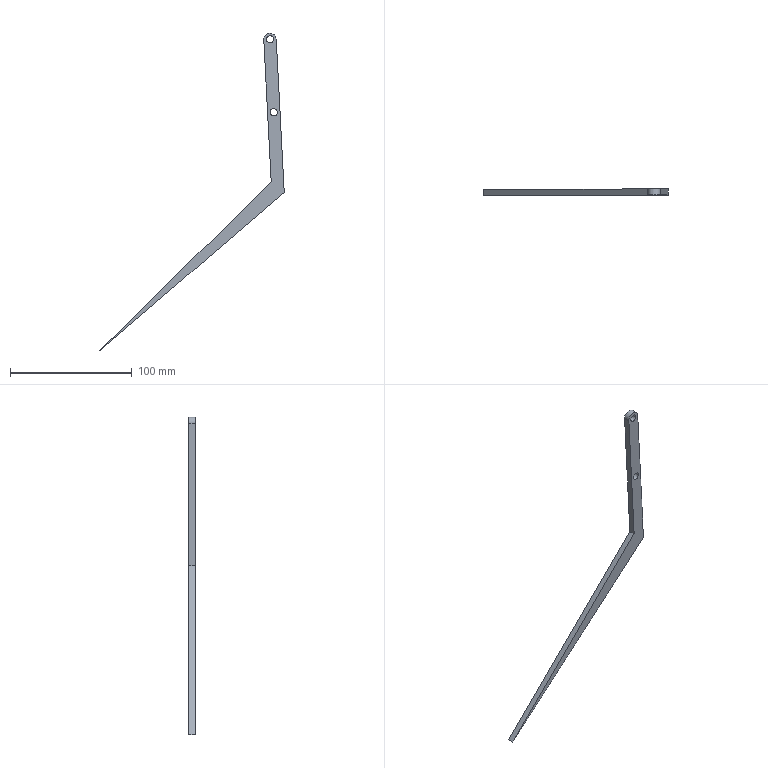Component | NX | 60 | 1 solid | 9 faces | box 151.75 x 5 x 261.36 mm | volume 12968 mm3 | plane 6 | cylinder 3 | commonest cylinder face diameters 5.929 x2 10.285 x1
STEP:
#1=CARTESIAN_POINT('',(0.,0.,0.));
#2=DIRECTION('',(0.,0.,1.));
#3=DIRECTION('',(1.,0.,0.));
#4=AXIS2_PLACEMENT_3D('',#1,#2,#3);
#5=CARTESIAN_POINT('',(-509.855,45.95,59.65));
#6=VERTEX_POINT('',#5);
#7=CARTESIAN_POINT('',(-499.584,45.95,60.187));
#8=VERTEX_POINT('',#7);
#9=CARTESIAN_POINT('',(-504.719,45.95,59.918));
#10=DIRECTION('',(0.,1.,0.));
#11=DIRECTION('',(-0.9986,0.,-0.05219));
#12=AXIS2_PLACEMENT_3D('',#9,#10,#11);
#13=CIRCLE('',#12,5.142);
#14=CARTESIAN_POINT('',(-504.719,40.95,59.918));
#15=DIRECTION('',(0.,1.,0.));
#16=DIRECTION('',(-0.9986,0.,-0.05219));
#17=AXIS2_PLACEMENT_3D('',#14,#15,#16);
#18=CYLINDRICAL_SURFACE('',#17,5.142);
#19=CARTESIAN_POINT('',(0.,5.));
#20=DIRECTION('',(1.,0.));
#21=VECTOR('',#20,1.);
#22=LINE('',#19,#21);
#23=(GEOMETRIC_REPRESENTATION_CONTEXT(2)PARAMETRIC_REPRESENTATION_CONTEXT()REPRESENTATION_CONTEXT('',''));
#24=DEFINITIONAL_REPRESENTATION('',(#22),#23);
#25=PCURVE('',#18,#24);
#26=CARTESIAN_POINT('',(-504.719,45.95,59.918));
#27=DIRECTION('',(0.,1.,0.));
#28=DIRECTION('',(-0.9986,0.,-0.05219));
#29=AXIS2_PLACEMENT_3D('',#26,#27,#28);
#30=PLANE('',#29);
#31=CARTESIAN_POINT('',(0.,0.));
#32=DIRECTION('',(1.,-0.));
#33=AXIS2_PLACEMENT_2D('',#31,#32);
#34=CIRCLE('',#33,5.142);
#35=(GEOMETRIC_REPRESENTATION_CONTEXT(2)PARAMETRIC_REPRESENTATION_CONTEXT()REPRESENTATION_CONTEXT('',''));
#36=DEFINITIONAL_REPRESENTATION('',(#34),#35);
#37=PCURVE('',#30,#36);
#38=SURFACE_CURVE('',#13,(#25,#37),.PCURVE_S1.);
#39=EDGE_CURVE('',#6,#8,#38,.T.);
#40=ORIENTED_EDGE('',*,*,#39,.F.);
#41=CARTESIAN_POINT('',(-509.855,40.95,59.65));
#42=VERTEX_POINT('',#41);
#43=CARTESIAN_POINT('',(-509.855,40.95,59.65));
#44=DIRECTION('',(0.,1.,0.));
#45=VECTOR('',#44,1.);
#46=LINE('',#43,#45);
#47=CARTESIAN_POINT('',(0.,0.));
#48=DIRECTION('',(0.,1.));
#49=VECTOR('',#48,1.);
#50=LINE('',#47,#49);
#51=(GEOMETRIC_REPRESENTATION_CONTEXT(2)PARAMETRIC_REPRESENTATION_CONTEXT()REPRESENTATION_CONTEXT('',''));
#52=DEFINITIONAL_REPRESENTATION('',(#50),#51);
#53=PCURVE('',#18,#52);
#54=CARTESIAN_POINT('',(-503.751,40.95,-57.127));
#55=DIRECTION('',(-0.9986,0.,-0.05219));
#56=DIRECTION('',(-0.05219,0.,0.9986));
#57=AXIS2_PLACEMENT_3D('',#54,#55,#56);
#58=PLANE('',#57);
#59=CARTESIAN_POINT('',(116.936,0.));
#60=DIRECTION('',(0.,1.));
#61=VECTOR('',#60,1.);
#62=LINE('',#59,#61);
#63=(GEOMETRIC_REPRESENTATION_CONTEXT(2)PARAMETRIC_REPRESENTATION_CONTEXT()REPRESENTATION_CONTEXT('',''));
#64=DEFINITIONAL_REPRESENTATION('',(#62),#63);
#65=PCURVE('',#58,#64);
#66=SURFACE_CURVE('',#46,(#53,#65),.PCURVE_S1.);
#67=EDGE_CURVE('',#42,#6,#66,.T.);
#68=ORIENTED_EDGE('',*,*,#67,.F.);
#69=CARTESIAN_POINT('',(-499.584,40.95,60.187));
#70=VERTEX_POINT('',#69);
#71=CARTESIAN_POINT('',(-504.719,40.95,59.918));
#72=DIRECTION('',(0.,1.,0.));
#73=DIRECTION('',(-0.9986,0.,-0.05219));
#74=AXIS2_PLACEMENT_3D('',#71,#72,#73);
#75=CIRCLE('',#74,5.142);
#76=CARTESIAN_POINT('',(0.,0.));
#77=DIRECTION('',(1.,0.));
#78=VECTOR('',#77,1.);
#79=LINE('',#76,#78);
#80=(GEOMETRIC_REPRESENTATION_CONTEXT(2)PARAMETRIC_REPRESENTATION_CONTEXT()REPRESENTATION_CONTEXT('',''));
#81=DEFINITIONAL_REPRESENTATION('',(#79),#80);
#82=PCURVE('',#18,#81);
#83=CARTESIAN_POINT('',(-504.719,40.95,59.918));
#84=DIRECTION('',(0.,1.,0.));
#85=DIRECTION('',(-0.9986,0.,-0.05219));
#86=AXIS2_PLACEMENT_3D('',#83,#84,#85);
#87=PLANE('',#86);
#88=CARTESIAN_POINT('',(0.,0.));
#89=DIRECTION('',(1.,-0.));
#90=AXIS2_PLACEMENT_2D('',#88,#89);
#91=CIRCLE('',#90,5.142);
#92=(GEOMETRIC_REPRESENTATION_CONTEXT(2)PARAMETRIC_REPRESENTATION_CONTEXT()REPRESENTATION_CONTEXT('',''));
#93=DEFINITIONAL_REPRESENTATION('',(#91),#92);
#94=PCURVE('',#87,#93);
#95=SURFACE_CURVE('',#75,(#82,#94),.PCURVE_S1.);
#96=EDGE_CURVE('',#42,#70,#95,.T.);
#97=ORIENTED_EDGE('',*,*,#96,.T.);
#98=CARTESIAN_POINT('',(-499.584,40.95,60.187));
#99=DIRECTION('',(0.,1.,0.));
#100=VECTOR('',#99,1.);
#101=LINE('',#98,#100);
#102=CARTESIAN_POINT('',(3.142,0.));
#103=DIRECTION('',(0.,1.));
#104=VECTOR('',#103,1.);
#105=LINE('',#102,#104);
#106=(GEOMETRIC_REPRESENTATION_CONTEXT(2)PARAMETRIC_REPRESENTATION_CONTEXT()REPRESENTATION_CONTEXT('',''));
#107=DEFINITIONAL_REPRESENTATION('',(#105),#106);
#108=PCURVE('',#18,#107);
#109=CARTESIAN_POINT('',(-496.452,40.95,0.2684));
#110=DIRECTION('',(0.9986,0.,0.05219));
#111=DIRECTION('',(0.05219,0.,-0.9986));
#112=AXIS2_PLACEMENT_3D('',#109,#110,#111);
#113=PLANE('',#112);
#114=CARTESIAN_POINT('',(-60.,0.));
#115=DIRECTION('',(0.,1.));
#116=VECTOR('',#115,1.);
#117=LINE('',#114,#116);
#118=(GEOMETRIC_REPRESENTATION_CONTEXT(2)PARAMETRIC_REPRESENTATION_CONTEXT()REPRESENTATION_CONTEXT('',''));
#119=DEFINITIONAL_REPRESENTATION('',(#117),#118);
#120=PCURVE('',#113,#119);
#121=SURFACE_CURVE('',#101,(#108,#120),.PCURVE_S1.);
#122=EDGE_CURVE('',#70,#8,#121,.T.);
#123=ORIENTED_EDGE('',*,*,#122,.T.);
#124=EDGE_LOOP('',(#40,#68,#97,#123));
#125=FACE_BOUND('',#124,.T.);
#126=ADVANCED_FACE('',(#125),#18,.T.);
#127=CARTESIAN_POINT('',(-493.001,45.95,-65.77));
#128=VERTEX_POINT('',#127);
#129=CARTESIAN_POINT('',(-496.452,45.95,0.2684));
#130=DIRECTION('',(0.05219,0.,-0.9986));
#131=VECTOR('',#130,1.);
#132=LINE('',#129,#131);
#133=CARTESIAN_POINT('',(0.,5.));
#134=DIRECTION('',(1.,0.));
#135=VECTOR('',#134,1.);
#136=LINE('',#133,#135);
#137=(GEOMETRIC_REPRESENTATION_CONTEXT(2)PARAMETRIC_REPRESENTATION_CONTEXT()REPRESENTATION_CONTEXT('',''));
#138=DEFINITIONAL_REPRESENTATION('',(#136),#137);
#139=PCURVE('',#113,#138);
#140=CARTESIAN_POINT('',(-5.142,-60.));
#141=DIRECTION('',(0.,-1.));
#142=VECTOR('',#141,1.);
#143=LINE('',#140,#142);
#144=(GEOMETRIC_REPRESENTATION_CONTEXT(2)PARAMETRIC_REPRESENTATION_CONTEXT()REPRESENTATION_CONTEXT('',''));
#145=DEFINITIONAL_REPRESENTATION('',(#143),#144);
#146=PCURVE('',#30,#145);
#147=SURFACE_CURVE('',#132,(#139,#146),.PCURVE_S1.);
#148=EDGE_CURVE('',#8,#128,#147,.T.);
#149=ORIENTED_EDGE('',*,*,#148,.F.);
#150=ORIENTED_EDGE('',*,*,#122,.F.);
#151=CARTESIAN_POINT('',(-493.001,40.95,-65.77));
#152=VERTEX_POINT('',#151);
#153=CARTESIAN_POINT('',(-499.584,40.95,60.187));
#154=DIRECTION('',(0.05219,0.,-0.9986));
#155=VECTOR('',#154,1.);
#156=LINE('',#153,#155);
#157=CARTESIAN_POINT('',(-60.,0.));
#158=DIRECTION('',(1.,0.));
#159=VECTOR('',#158,1.);
#160=LINE('',#157,#159);
#161=(GEOMETRIC_REPRESENTATION_CONTEXT(2)PARAMETRIC_REPRESENTATION_CONTEXT()REPRESENTATION_CONTEXT('',''));
#162=DEFINITIONAL_REPRESENTATION('',(#160),#161);
#163=PCURVE('',#113,#162);
#164=CARTESIAN_POINT('',(-5.142,0.));
#165=DIRECTION('',(0.,-1.));
#166=VECTOR('',#165,1.);
#167=LINE('',#164,#166);
#168=(GEOMETRIC_REPRESENTATION_CONTEXT(2)PARAMETRIC_REPRESENTATION_CONTEXT()REPRESENTATION_CONTEXT('',''));
#169=DEFINITIONAL_REPRESENTATION('',(#167),#168);
#170=PCURVE('',#87,#169);
#171=SURFACE_CURVE('',#156,(#163,#170),.PCURVE_S1.);
#172=EDGE_CURVE('',#70,#152,#171,.T.);
#173=ORIENTED_EDGE('',*,*,#172,.T.);
#174=CARTESIAN_POINT('',(-493.001,40.95,-65.77));
#175=DIRECTION('',(0.,1.,0.));
#176=VECTOR('',#175,1.);
#177=LINE('',#174,#176);
#178=CARTESIAN_POINT('',(66.128,0.));
#179=DIRECTION('',(0.,1.));
#180=VECTOR('',#179,1.);
#181=LINE('',#178,#180);
#182=(GEOMETRIC_REPRESENTATION_CONTEXT(2)PARAMETRIC_REPRESENTATION_CONTEXT()REPRESENTATION_CONTEXT('',''));
#183=DEFINITIONAL_REPRESENTATION('',(#181),#182);
#184=PCURVE('',#113,#183);
#185=CARTESIAN_POINT('',(-493.001,40.95,-65.77));
#186=DIRECTION('',(0.6521,0.,-0.7581));
#187=DIRECTION('',(-0.7581,0.,-0.6521));
#188=AXIS2_PLACEMENT_3D('',#185,#186,#187);
#189=PLANE('',#188);
#190=CARTESIAN_POINT('',(0.,0.));
#191=DIRECTION('',(0.,1.));
#192=VECTOR('',#191,1.);
#193=LINE('',#190,#192);
#194=(GEOMETRIC_REPRESENTATION_CONTEXT(2)PARAMETRIC_REPRESENTATION_CONTEXT()REPRESENTATION_CONTEXT('',''));
#195=DEFINITIONAL_REPRESENTATION('',(#193),#194);
#196=PCURVE('',#189,#195);
#197=SURFACE_CURVE('',#177,(#184,#196),.PCURVE_S1.);
#198=EDGE_CURVE('',#152,#128,#197,.T.);
#199=ORIENTED_EDGE('',*,*,#198,.T.);
#200=EDGE_LOOP('',(#149,#150,#173,#199));
#201=FACE_BOUND('',#200,.T.);
#202=ADVANCED_FACE('',(#201),#113,.T.);
#203=CARTESIAN_POINT('',(-644.746,45.95,-196.297));
#204=VERTEX_POINT('',#203);
#205=CARTESIAN_POINT('',(-493.001,45.95,-65.77));
#206=DIRECTION('',(-0.7581,0.,-0.6521));
#207=VECTOR('',#206,1.);
#208=LINE('',#205,#207);
#209=CARTESIAN_POINT('',(0.,5.));
#210=DIRECTION('',(1.,0.));
#211=VECTOR('',#210,1.);
#212=LINE('',#209,#211);
#213=(GEOMETRIC_REPRESENTATION_CONTEXT(2)PARAMETRIC_REPRESENTATION_CONTEXT()REPRESENTATION_CONTEXT('',''));
#214=DEFINITIONAL_REPRESENTATION('',(#212),#213);
#215=PCURVE('',#189,#214);
#216=CARTESIAN_POINT('',(-5.142,-126.128));
#217=DIRECTION('',(0.7911,-0.6117));
#218=VECTOR('',#217,1.);
#219=LINE('',#216,#218);
#220=(GEOMETRIC_REPRESENTATION_CONTEXT(2)PARAMETRIC_REPRESENTATION_CONTEXT()REPRESENTATION_CONTEXT('',''));
#221=DEFINITIONAL_REPRESENTATION('',(#219),#220);
#222=PCURVE('',#30,#221);
#223=SURFACE_CURVE('',#208,(#215,#222),.PCURVE_S1.);
#224=EDGE_CURVE('',#128,#204,#223,.T.);
#225=ORIENTED_EDGE('',*,*,#224,.F.);
#226=ORIENTED_EDGE('',*,*,#198,.F.);
#227=CARTESIAN_POINT('',(-644.746,40.95,-196.297));
#228=VERTEX_POINT('',#227);
#229=CARTESIAN_POINT('',(-493.001,40.95,-65.77));
#230=DIRECTION('',(-0.7581,0.,-0.6521));
#231=VECTOR('',#230,1.);
#232=LINE('',#229,#231);
#233=CARTESIAN_POINT('',(0.,0.));
#234=DIRECTION('',(1.,0.));
#235=VECTOR('',#234,1.);
#236=LINE('',#233,#235);
#237=(GEOMETRIC_REPRESENTATION_CONTEXT(2)PARAMETRIC_REPRESENTATION_CONTEXT()REPRESENTATION_CONTEXT('',''));
#238=DEFINITIONAL_REPRESENTATION('',(#236),#237);
#239=PCURVE('',#189,#238);
#240=CARTESIAN_POINT('',(-5.142,-126.128));
#241=DIRECTION('',(0.7911,-0.6117));
#242=VECTOR('',#241,1.);
#243=LINE('',#240,#242);
#244=(GEOMETRIC_REPRESENTATION_CONTEXT(2)PARAMETRIC_REPRESENTATION_CONTEXT()REPRESENTATION_CONTEXT('',''));
#245=DEFINITIONAL_REPRESENTATION('',(#243),#244);
#246=PCURVE('',#87,#245);
#247=SURFACE_CURVE('',#232,(#239,#246),.PCURVE_S1.);
#248=EDGE_CURVE('',#152,#228,#247,.T.);
#249=ORIENTED_EDGE('',*,*,#248,.T.);
#250=CARTESIAN_POINT('',(-644.746,40.95,-196.297));
#251=DIRECTION('',(0.,1.,0.));
#252=VECTOR('',#251,1.);
#253=LINE('',#250,#252);
#254=CARTESIAN_POINT('',(200.16,0.));
#255=DIRECTION('',(0.,1.));
#256=VECTOR('',#255,1.);
#257=LINE('',#254,#256);
#258=(GEOMETRIC_REPRESENTATION_CONTEXT(2)PARAMETRIC_REPRESENTATION_CONTEXT()REPRESENTATION_CONTEXT('',''));
#259=DEFINITIONAL_REPRESENTATION('',(#257),#258);
#260=PCURVE('',#189,#259);
#261=CARTESIAN_POINT('',(-644.746,40.95,-196.297));
#262=DIRECTION('',(-0.7025,0.,0.7117));
#263=DIRECTION('',(0.7117,0.,0.7025));
#264=AXIS2_PLACEMENT_3D('',#261,#262,#263);
#265=PLANE('',#264);
#266=CARTESIAN_POINT('',(0.,0.));
#267=DIRECTION('',(0.,1.));
#268=VECTOR('',#267,1.);
#269=LINE('',#266,#268);
#270=(GEOMETRIC_REPRESENTATION_CONTEXT(2)PARAMETRIC_REPRESENTATION_CONTEXT()REPRESENTATION_CONTEXT('',''));
#271=DEFINITIONAL_REPRESENTATION('',(#269),#270);
#272=PCURVE('',#265,#271);
#273=SURFACE_CURVE('',#253,(#260,#272),.PCURVE_S1.);
#274=EDGE_CURVE('',#228,#204,#273,.T.);
#275=ORIENTED_EDGE('',*,*,#274,.T.);
#276=EDGE_LOOP('',(#225,#226,#249,#275));
#277=FACE_BOUND('',#276,.T.);
#278=ADVANCED_FACE('',(#277),#189,.T.);
#279=CARTESIAN_POINT('',(-503.751,45.95,-57.127));
#280=VERTEX_POINT('',#279);
#281=CARTESIAN_POINT('',(-644.746,45.95,-196.297));
#282=DIRECTION('',(0.7117,0.,0.7025));
#283=VECTOR('',#282,1.);
#284=LINE('',#281,#283);
#285=CARTESIAN_POINT('',(0.,5.));
#286=DIRECTION('',(1.,0.));
#287=VECTOR('',#286,1.);
#288=LINE('',#285,#287);
#289=(GEOMETRIC_REPRESENTATION_CONTEXT(2)PARAMETRIC_REPRESENTATION_CONTEXT()REPRESENTATION_CONTEXT('',''));
#290=DEFINITIONAL_REPRESENTATION('',(#288),#289);
#291=PCURVE('',#265,#290);
#292=CARTESIAN_POINT('',(153.209,-248.558));
#293=DIRECTION('',(-0.7474,0.6644));
#294=VECTOR('',#293,1.);
#295=LINE('',#292,#294);
#296=(GEOMETRIC_REPRESENTATION_CONTEXT(2)PARAMETRIC_REPRESENTATION_CONTEXT()REPRESENTATION_CONTEXT('',''));
#297=DEFINITIONAL_REPRESENTATION('',(#295),#296);
#298=PCURVE('',#30,#297);
#299=SURFACE_CURVE('',#284,(#291,#298),.PCURVE_S1.);
#300=EDGE_CURVE('',#204,#280,#299,.T.);
#301=ORIENTED_EDGE('',*,*,#300,.F.);
#302=ORIENTED_EDGE('',*,*,#274,.F.);
#303=CARTESIAN_POINT('',(-503.751,40.95,-57.127));
#304=VERTEX_POINT('',#303);
#305=CARTESIAN_POINT('',(-644.746,40.95,-196.297));
#306=DIRECTION('',(0.7117,0.,0.7025));
#307=VECTOR('',#306,1.);
#308=LINE('',#305,#307);
#309=CARTESIAN_POINT('',(0.,0.));
#310=DIRECTION('',(1.,0.));
#311=VECTOR('',#310,1.);
#312=LINE('',#309,#311);
#313=(GEOMETRIC_REPRESENTATION_CONTEXT(2)PARAMETRIC_REPRESENTATION_CONTEXT()REPRESENTATION_CONTEXT('',''));
#314=DEFINITIONAL_REPRESENTATION('',(#312),#313);
#315=PCURVE('',#265,#314);
#316=CARTESIAN_POINT('',(153.209,-248.558));
#317=DIRECTION('',(-0.7474,0.6644));
#318=VECTOR('',#317,1.);
#319=LINE('',#316,#318);
#320=(GEOMETRIC_REPRESENTATION_CONTEXT(2)PARAMETRIC_REPRESENTATION_CONTEXT()REPRESENTATION_CONTEXT('',''));
#321=DEFINITIONAL_REPRESENTATION('',(#319),#320);
#322=PCURVE('',#87,#321);
#323=SURFACE_CURVE('',#308,(#315,#322),.PCURVE_S1.);
#324=EDGE_CURVE('',#228,#304,#323,.T.);
#325=ORIENTED_EDGE('',*,*,#324,.T.);
#326=CARTESIAN_POINT('',(-503.751,40.95,-57.127));
#327=DIRECTION('',(0.,1.,0.));
#328=VECTOR('',#327,1.);
#329=LINE('',#326,#328);
#330=CARTESIAN_POINT('',(198.111,0.));
#331=DIRECTION('',(0.,1.));
#332=VECTOR('',#331,1.);
#333=LINE('',#330,#332);
#334=(GEOMETRIC_REPRESENTATION_CONTEXT(2)PARAMETRIC_REPRESENTATION_CONTEXT()REPRESENTATION_CONTEXT('',''));
#335=DEFINITIONAL_REPRESENTATION('',(#333),#334);
#336=PCURVE('',#265,#335);
#337=CARTESIAN_POINT('',(0.,0.));
#338=DIRECTION('',(0.,1.));
#339=VECTOR('',#338,1.);
#340=LINE('',#337,#339);
#341=(GEOMETRIC_REPRESENTATION_CONTEXT(2)PARAMETRIC_REPRESENTATION_CONTEXT()REPRESENTATION_CONTEXT('',''));
#342=DEFINITIONAL_REPRESENTATION('',(#340),#341);
#343=PCURVE('',#58,#342);
#344=SURFACE_CURVE('',#329,(#336,#343),.PCURVE_S1.);
#345=EDGE_CURVE('',#304,#280,#344,.T.);
#346=ORIENTED_EDGE('',*,*,#345,.T.);
#347=EDGE_LOOP('',(#301,#302,#325,#346));
#348=FACE_BOUND('',#347,.T.);
#349=ADVANCED_FACE('',(#348),#265,.T.);
#350=CARTESIAN_POINT('',(-504.548,40.95,-0.1547));
#351=VERTEX_POINT('',#350);
#352=CARTESIAN_POINT('',(-501.588,40.95,0.));
#353=DIRECTION('',(0.,1.,0.));
#354=DIRECTION('',(-0.9986,0.,-0.05219));
#355=AXIS2_PLACEMENT_3D('',#352,#353,#354);
#356=CIRCLE('',#355,2.964);
#357=CARTESIAN_POINT('',(-501.588,40.95,0.));
#358=DIRECTION('',(0.,1.,0.));
#359=DIRECTION('',(-0.9986,0.,-0.05219));
#360=AXIS2_PLACEMENT_3D('',#357,#358,#359);
#361=CYLINDRICAL_SURFACE('',#360,2.964);
#362=CARTESIAN_POINT('',(0.,0.));
#363=DIRECTION('',(1.,0.));
#364=VECTOR('',#363,1.);
#365=LINE('',#362,#364);
#366=(GEOMETRIC_REPRESENTATION_CONTEXT(2)PARAMETRIC_REPRESENTATION_CONTEXT()REPRESENTATION_CONTEXT('',''));
#367=DEFINITIONAL_REPRESENTATION('',(#365),#366);
#368=PCURVE('',#361,#367);
#369=CARTESIAN_POINT('',(-0.,-60.));
#370=DIRECTION('',(1.,0.));
#371=AXIS2_PLACEMENT_2D('',#369,#370);
#372=CIRCLE('',#371,2.964);
#373=(GEOMETRIC_REPRESENTATION_CONTEXT(2)PARAMETRIC_REPRESENTATION_CONTEXT()REPRESENTATION_CONTEXT('',''));
#374=DEFINITIONAL_REPRESENTATION('',(#372),#373);
#375=PCURVE('',#87,#374);
#376=SURFACE_CURVE('',#356,(#368,#375),.PCURVE_S1.);
#377=EDGE_CURVE('',#351,#351,#376,.T.);
#378=ORIENTED_EDGE('',*,*,#377,.T.);
#379=CARTESIAN_POINT('',(-504.548,45.95,-0.1547));
#380=VERTEX_POINT('',#379);
#381=CARTESIAN_POINT('',(-504.548,40.95,-0.1547));
#382=CARTESIAN_POINT('',(-504.548,45.95,-0.1547));
#383=B_SPLINE_CURVE_WITH_KNOTS('',1,(#381,#382),.UNSPECIFIED.,.F.,.F.,(2,2),(0.,5.),.PIECEWISE_BEZIER_KNOTS.);
#384=CARTESIAN_POINT('',(6.283,0.));
#385=DIRECTION('',(0.,1.));
#386=VECTOR('',#385,1.);
#387=LINE('',#384,#386);
#388=(GEOMETRIC_REPRESENTATION_CONTEXT(2)PARAMETRIC_REPRESENTATION_CONTEXT()REPRESENTATION_CONTEXT('',''));
#389=DEFINITIONAL_REPRESENTATION('',(#387),#388);
#390=PCURVE('',#361,#389);
#391=CARTESIAN_POINT('',(0.,0.));
#392=DIRECTION('',(0.,1.));
#393=VECTOR('',#392,1.);
#394=LINE('',#391,#393);
#395=(GEOMETRIC_REPRESENTATION_CONTEXT(2)PARAMETRIC_REPRESENTATION_CONTEXT()REPRESENTATION_CONTEXT('',''));
#396=DEFINITIONAL_REPRESENTATION('',(#394),#395);
#397=PCURVE('',#361,#396);
#398=SEAM_CURVE('',#383,(#390,#397),.PCURVE_S1.);
#399=EDGE_CURVE('',#351,#380,#398,.T.);
#400=ORIENTED_EDGE('',*,*,#399,.T.);
#401=CARTESIAN_POINT('',(-501.588,45.95,0.));
#402=DIRECTION('',(0.,1.,0.));
#403=DIRECTION('',(-0.9986,0.,-0.05219));
#404=AXIS2_PLACEMENT_3D('',#401,#402,#403);
#405=CIRCLE('',#404,2.964);
#406=CARTESIAN_POINT('',(0.,5.));
#407=DIRECTION('',(1.,0.));
#408=VECTOR('',#407,1.);
#409=LINE('',#406,#408);
#410=(GEOMETRIC_REPRESENTATION_CONTEXT(2)PARAMETRIC_REPRESENTATION_CONTEXT()REPRESENTATION_CONTEXT('',''));
#411=DEFINITIONAL_REPRESENTATION('',(#409),#410);
#412=PCURVE('',#361,#411);
#413=CARTESIAN_POINT('',(-0.,-60.));
#414=DIRECTION('',(1.,0.));
#415=AXIS2_PLACEMENT_2D('',#413,#414);
#416=CIRCLE('',#415,2.964);
#417=(GEOMETRIC_REPRESENTATION_CONTEXT(2)PARAMETRIC_REPRESENTATION_CONTEXT()REPRESENTATION_CONTEXT('',''));
#418=DEFINITIONAL_REPRESENTATION('',(#416),#417);
#419=PCURVE('',#30,#418);
#420=SURFACE_CURVE('',#405,(#412,#419),.PCURVE_S1.);
#421=EDGE_CURVE('',#380,#380,#420,.T.);
#422=ORIENTED_EDGE('',*,*,#421,.F.);
#423=ORIENTED_EDGE('',*,*,#399,.F.);
#424=EDGE_LOOP('',(#378,#400,#422,#423));
#425=FACE_BOUND('',#424,.F.);
#426=ADVANCED_FACE('',(#425),#361,.F.);
#427=CARTESIAN_POINT('',(-503.751,45.95,-57.127));
#428=DIRECTION('',(-0.05219,0.,0.9986));
#429=VECTOR('',#428,1.);
#430=LINE('',#427,#429);
#431=CARTESIAN_POINT('',(0.,5.));
#432=DIRECTION('',(1.,0.));
#433=VECTOR('',#432,1.);
#434=LINE('',#431,#433);
#435=(GEOMETRIC_REPRESENTATION_CONTEXT(2)PARAMETRIC_REPRESENTATION_CONTEXT()REPRESENTATION_CONTEXT('',''));
#436=DEFINITIONAL_REPRESENTATION('',(#434),#435);
#437=PCURVE('',#58,#436);
#438=CARTESIAN_POINT('',(5.142,-116.936));
#439=DIRECTION('',(-0.,1.));
#440=VECTOR('',#439,1.);
#441=LINE('',#438,#440);
#442=(GEOMETRIC_REPRESENTATION_CONTEXT(2)PARAMETRIC_REPRESENTATION_CONTEXT()REPRESENTATION_CONTEXT('',''));
#443=DEFINITIONAL_REPRESENTATION('',(#441),#442);
#444=PCURVE('',#30,#443);
#445=SURFACE_CURVE('',#430,(#437,#444),.PCURVE_S1.);
#446=EDGE_CURVE('',#280,#6,#445,.T.);
#447=ORIENTED_EDGE('',*,*,#446,.F.);
#448=ORIENTED_EDGE('',*,*,#345,.F.);
#449=CARTESIAN_POINT('',(-506.723,40.95,-0.2684));
#450=DIRECTION('',(-0.05219,0.,0.9986));
#451=VECTOR('',#450,1.);
#452=LINE('',#449,#451);
#453=CARTESIAN_POINT('',(56.936,0.));
#454=DIRECTION('',(1.,0.));
#455=VECTOR('',#454,1.);
#456=LINE('',#453,#455);
#457=(GEOMETRIC_REPRESENTATION_CONTEXT(2)PARAMETRIC_REPRESENTATION_CONTEXT()REPRESENTATION_CONTEXT('',''));
#458=DEFINITIONAL_REPRESENTATION('',(#456),#457);
#459=PCURVE('',#58,#458);
#460=CARTESIAN_POINT('',(5.142,-60.));
#461=DIRECTION('',(-0.,1.));
#462=VECTOR('',#461,1.);
#463=LINE('',#460,#462);
#464=(GEOMETRIC_REPRESENTATION_CONTEXT(2)PARAMETRIC_REPRESENTATION_CONTEXT()REPRESENTATION_CONTEXT('',''));
#465=DEFINITIONAL_REPRESENTATION('',(#463),#464);
#466=PCURVE('',#87,#465);
#467=SURFACE_CURVE('',#452,(#459,#466),.PCURVE_S1.);
#468=EDGE_CURVE('',#304,#42,#467,.T.);
#469=ORIENTED_EDGE('',*,*,#468,.T.);
#470=ORIENTED_EDGE('',*,*,#67,.T.);
#471=EDGE_LOOP('',(#447,#448,#469,#470));
#472=FACE_BOUND('',#471,.T.);
#473=ADVANCED_FACE('',(#472),#58,.T.);
#474=CARTESIAN_POINT('',(-507.679,40.95,59.764));
#475=VERTEX_POINT('',#474);
#476=CARTESIAN_POINT('',(-504.719,40.95,59.918));
#477=DIRECTION('',(0.,1.,0.));
#478=DIRECTION('',(-0.9986,0.,-0.05219));
#479=AXIS2_PLACEMENT_3D('',#476,#477,#478);
#480=CIRCLE('',#479,2.964);
#481=CARTESIAN_POINT('',(-504.719,40.95,59.918));
#482=DIRECTION('',(0.,1.,0.));
#483=DIRECTION('',(-0.9986,0.,-0.05219));
#484=AXIS2_PLACEMENT_3D('',#481,#482,#483);
#485=CYLINDRICAL_SURFACE('',#484,2.964);
#486=CARTESIAN_POINT('',(0.,0.));
#487=DIRECTION('',(1.,0.));
#488=VECTOR('',#487,1.);
#489=LINE('',#486,#488);
#490=(GEOMETRIC_REPRESENTATION_CONTEXT(2)PARAMETRIC_REPRESENTATION_CONTEXT()REPRESENTATION_CONTEXT('',''));
#491=DEFINITIONAL_REPRESENTATION('',(#489),#490);
#492=PCURVE('',#485,#491);
#493=CARTESIAN_POINT('',(0.,0.));
#494=DIRECTION('',(1.,-0.));
#495=AXIS2_PLACEMENT_2D('',#493,#494);
#496=CIRCLE('',#495,2.964);
#497=(GEOMETRIC_REPRESENTATION_CONTEXT(2)PARAMETRIC_REPRESENTATION_CONTEXT()REPRESENTATION_CONTEXT('',''));
#498=DEFINITIONAL_REPRESENTATION('',(#496),#497);
#499=PCURVE('',#87,#498);
#500=SURFACE_CURVE('',#480,(#492,#499),.PCURVE_S1.);
#501=EDGE_CURVE('',#475,#475,#500,.T.);
#502=ORIENTED_EDGE('',*,*,#501,.T.);
#503=CARTESIAN_POINT('',(-507.679,45.95,59.764));
#504=VERTEX_POINT('',#503);
#505=CARTESIAN_POINT('',(-507.679,40.95,59.764));
#506=CARTESIAN_POINT('',(-507.679,45.95,59.764));
#507=B_SPLINE_CURVE_WITH_KNOTS('',1,(#505,#506),.UNSPECIFIED.,.F.,.F.,(2,2),(0.,5.),.PIECEWISE_BEZIER_KNOTS.);
#508=CARTESIAN_POINT('',(6.283,0.));
#509=DIRECTION('',(0.,1.));
#510=VECTOR('',#509,1.);
#511=LINE('',#508,#510);
#512=(GEOMETRIC_REPRESENTATION_CONTEXT(2)PARAMETRIC_REPRESENTATION_CONTEXT()REPRESENTATION_CONTEXT('',''));
#513=DEFINITIONAL_REPRESENTATION('',(#511),#512);
#514=PCURVE('',#485,#513);
#515=CARTESIAN_POINT('',(0.,0.));
#516=DIRECTION('',(0.,1.));
#517=VECTOR('',#516,1.);
#518=LINE('',#515,#517);
#519=(GEOMETRIC_REPRESENTATION_CONTEXT(2)PARAMETRIC_REPRESENTATION_CONTEXT()REPRESENTATION_CONTEXT('',''));
#520=DEFINITIONAL_REPRESENTATION('',(#518),#519);
#521=PCURVE('',#485,#520);
#522=SEAM_CURVE('',#507,(#514,#521),.PCURVE_S1.);
#523=EDGE_CURVE('',#475,#504,#522,.T.);
#524=ORIENTED_EDGE('',*,*,#523,.T.);
#525=CARTESIAN_POINT('',(-504.719,45.95,59.918));
#526=DIRECTION('',(0.,1.,0.));
#527=DIRECTION('',(-0.9986,0.,-0.05219));
#528=AXIS2_PLACEMENT_3D('',#525,#526,#527);
#529=CIRCLE('',#528,2.964);
#530=CARTESIAN_POINT('',(0.,5.));
#531=DIRECTION('',(1.,0.));
#532=VECTOR('',#531,1.);
#533=LINE('',#530,#532);
#534=(GEOMETRIC_REPRESENTATION_CONTEXT(2)PARAMETRIC_REPRESENTATION_CONTEXT()REPRESENTATION_CONTEXT('',''));
#535=DEFINITIONAL_REPRESENTATION('',(#533),#534);
#536=PCURVE('',#485,#535);
#537=CARTESIAN_POINT('',(0.,0.));
#538=DIRECTION('',(1.,-0.));
#539=AXIS2_PLACEMENT_2D('',#537,#538);
#540=CIRCLE('',#539,2.964);
#541=(GEOMETRIC_REPRESENTATION_CONTEXT(2)PARAMETRIC_REPRESENTATION_CONTEXT()REPRESENTATION_CONTEXT('',''));
#542=DEFINITIONAL_REPRESENTATION('',(#540),#541);
#543=PCURVE('',#30,#542);
#544=SURFACE_CURVE('',#529,(#536,#543),.PCURVE_S1.);
#545=EDGE_CURVE('',#504,#504,#544,.T.);
#546=ORIENTED_EDGE('',*,*,#545,.F.);
#547=ORIENTED_EDGE('',*,*,#523,.F.);
#548=EDGE_LOOP('',(#502,#524,#546,#547));
#549=FACE_BOUND('',#548,.F.);
#550=ADVANCED_FACE('',(#549),#485,.F.);
#551=ORIENTED_EDGE('',*,*,#468,.F.);
#552=ORIENTED_EDGE('',*,*,#324,.F.);
#553=ORIENTED_EDGE('',*,*,#248,.F.);
#554=ORIENTED_EDGE('',*,*,#172,.F.);
#555=ORIENTED_EDGE('',*,*,#96,.F.);
#556=EDGE_LOOP('',(#551,#552,#553,#554,#555));
#557=FACE_BOUND('',#556,.T.);
#558=ORIENTED_EDGE('',*,*,#377,.T.);
#559=EDGE_LOOP('',(#558));
#560=FACE_BOUND('',#559,.T.);
#561=ORIENTED_EDGE('',*,*,#501,.T.);
#562=EDGE_LOOP('',(#561));
#563=FACE_BOUND('',#562,.T.);
#564=ADVANCED_FACE('',(#557,#560,#563),#87,.F.);
#565=ORIENTED_EDGE('',*,*,#446,.T.);
#566=ORIENTED_EDGE('',*,*,#39,.T.);
#567=ORIENTED_EDGE('',*,*,#148,.T.);
#568=ORIENTED_EDGE('',*,*,#224,.T.);
#569=ORIENTED_EDGE('',*,*,#300,.T.);
#570=EDGE_LOOP('',(#565,#566,#567,#568,#569));
#571=FACE_BOUND('',#570,.T.);
#572=ORIENTED_EDGE('',*,*,#421,.F.);
#573=EDGE_LOOP('',(#572));
#574=FACE_BOUND('',#573,.T.);
#575=ORIENTED_EDGE('',*,*,#545,.F.);
#576=EDGE_LOOP('',(#575));
#577=FACE_BOUND('',#576,.T.);
#578=ADVANCED_FACE('',(#571,#574,#577),#30,.T.);
#579=CLOSED_SHELL('',(#126,#202,#278,#349,#426,#473,#550,#564,#578));
#580=MANIFOLD_SOLID_BREP('',#579);
#581=(LENGTH_UNIT()NAMED_UNIT(*)SI_UNIT(.MILLI.,.METRE.));
#582=UNCERTAINTY_MEASURE_WITH_UNIT(LENGTH_MEASURE(0.000002),#581,'','');
#583=(NAMED_UNIT(*)PLANE_ANGLE_UNIT()SI_UNIT($,.RADIAN.));
#584=(NAMED_UNIT(*)SI_UNIT($,.STERADIAN.)SOLID_ANGLE_UNIT());
#585=(GEOMETRIC_REPRESENTATION_CONTEXT(3)GLOBAL_UNCERTAINTY_ASSIGNED_CONTEXT((#582))GLOBAL_UNIT_ASSIGNED_CONTEXT((#581,#583,#584))REPRESENTATION_CONTEXT('',''));
#586=ADVANCED_BREP_SHAPE_REPRESENTATION('',(#4,#580),#585);